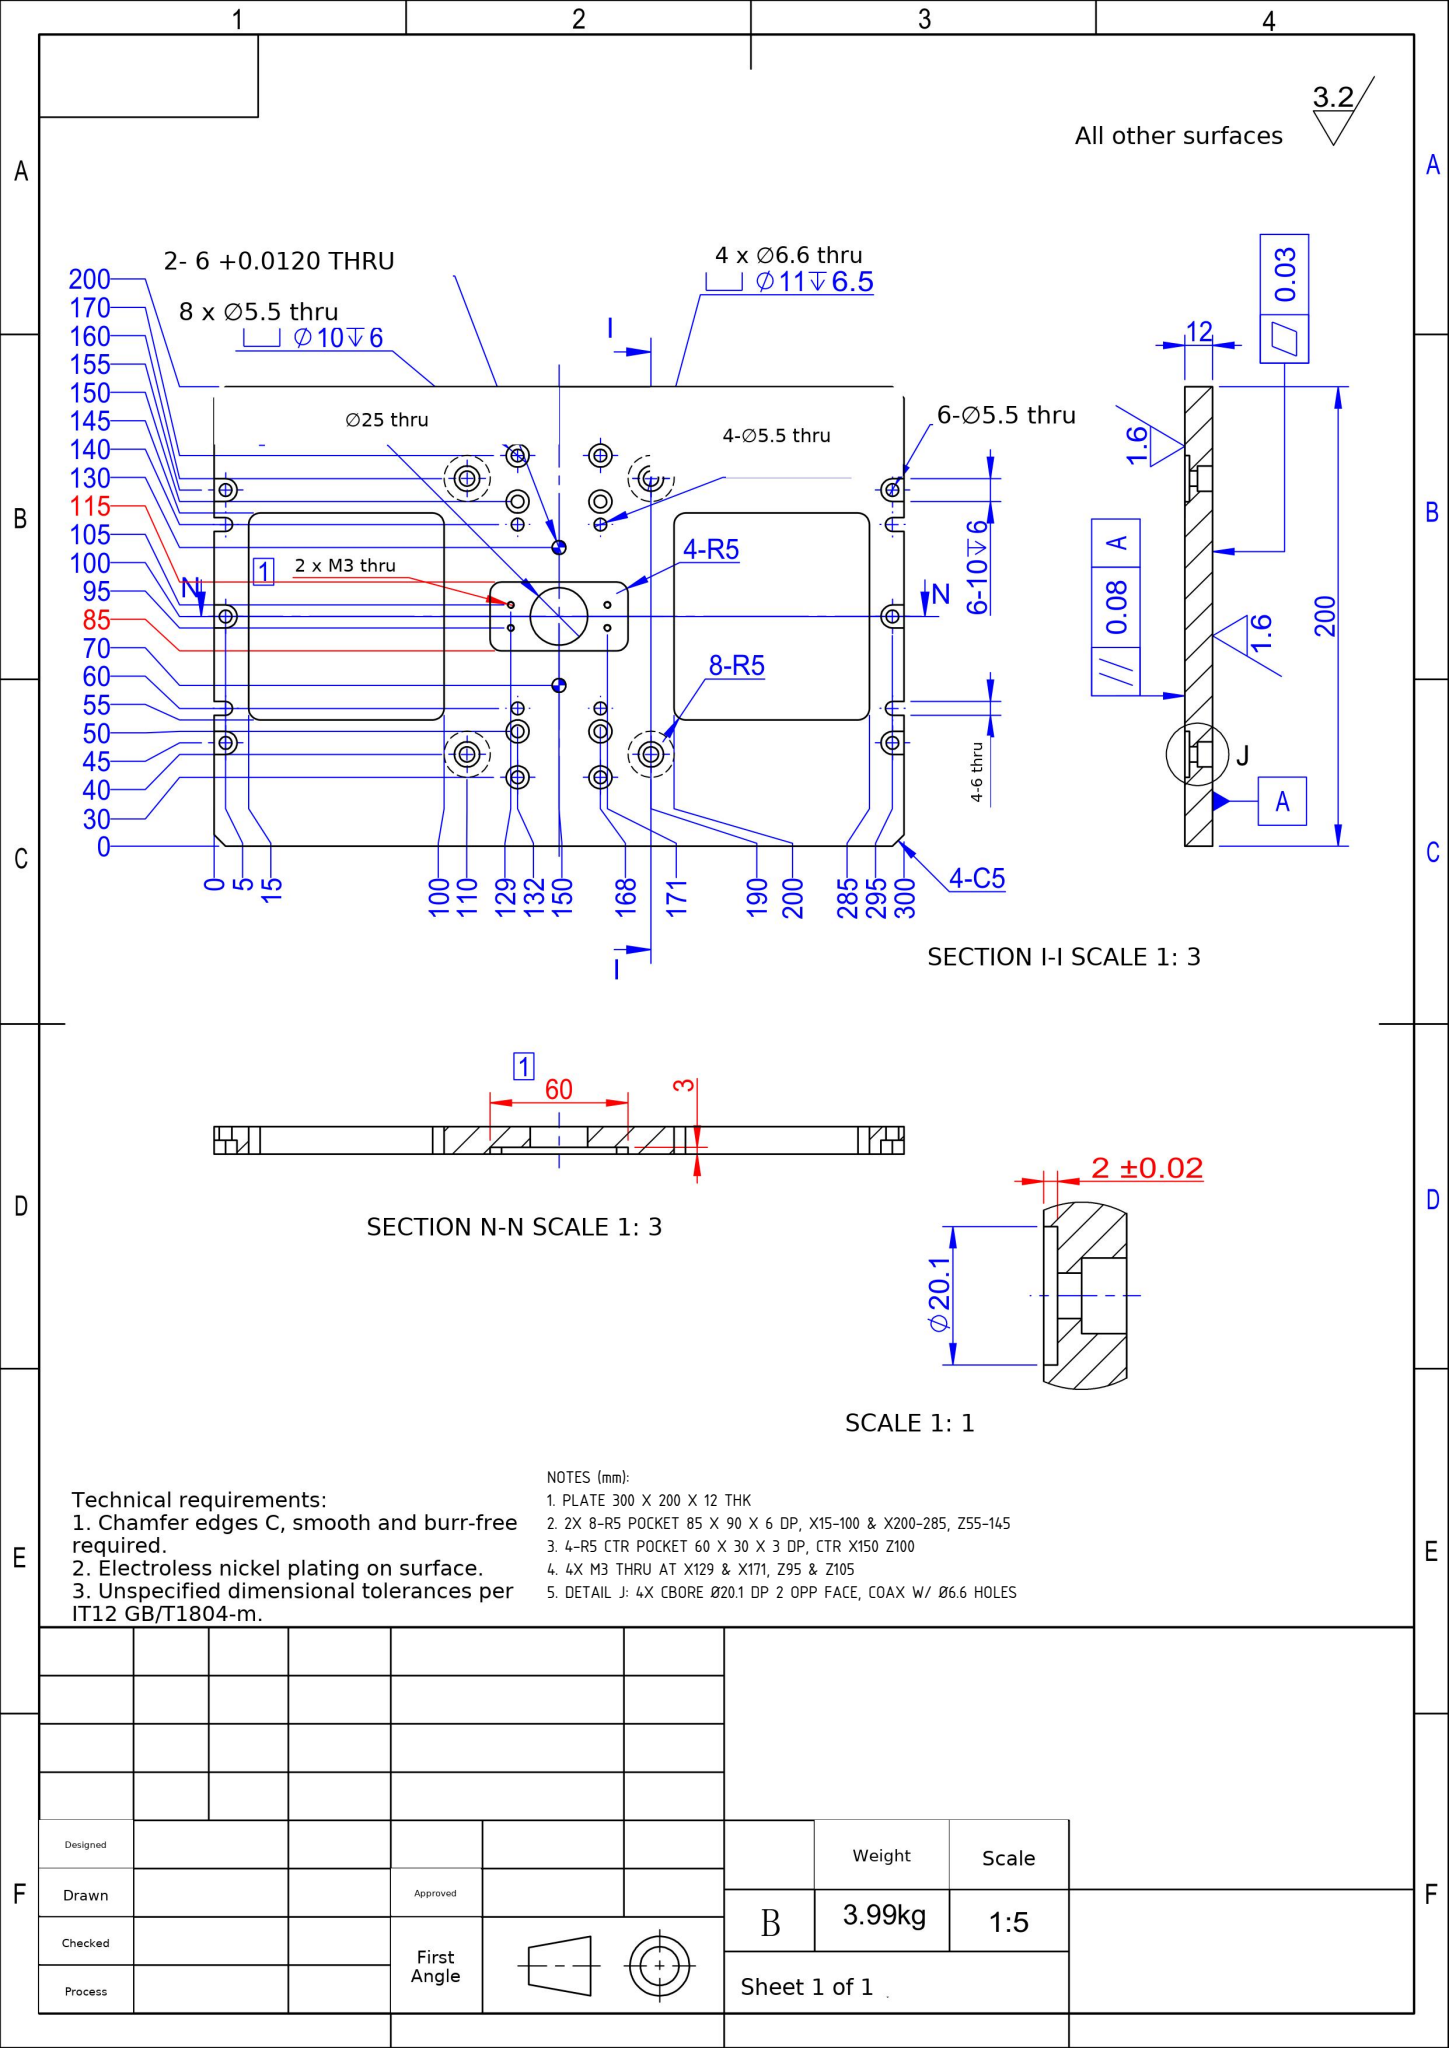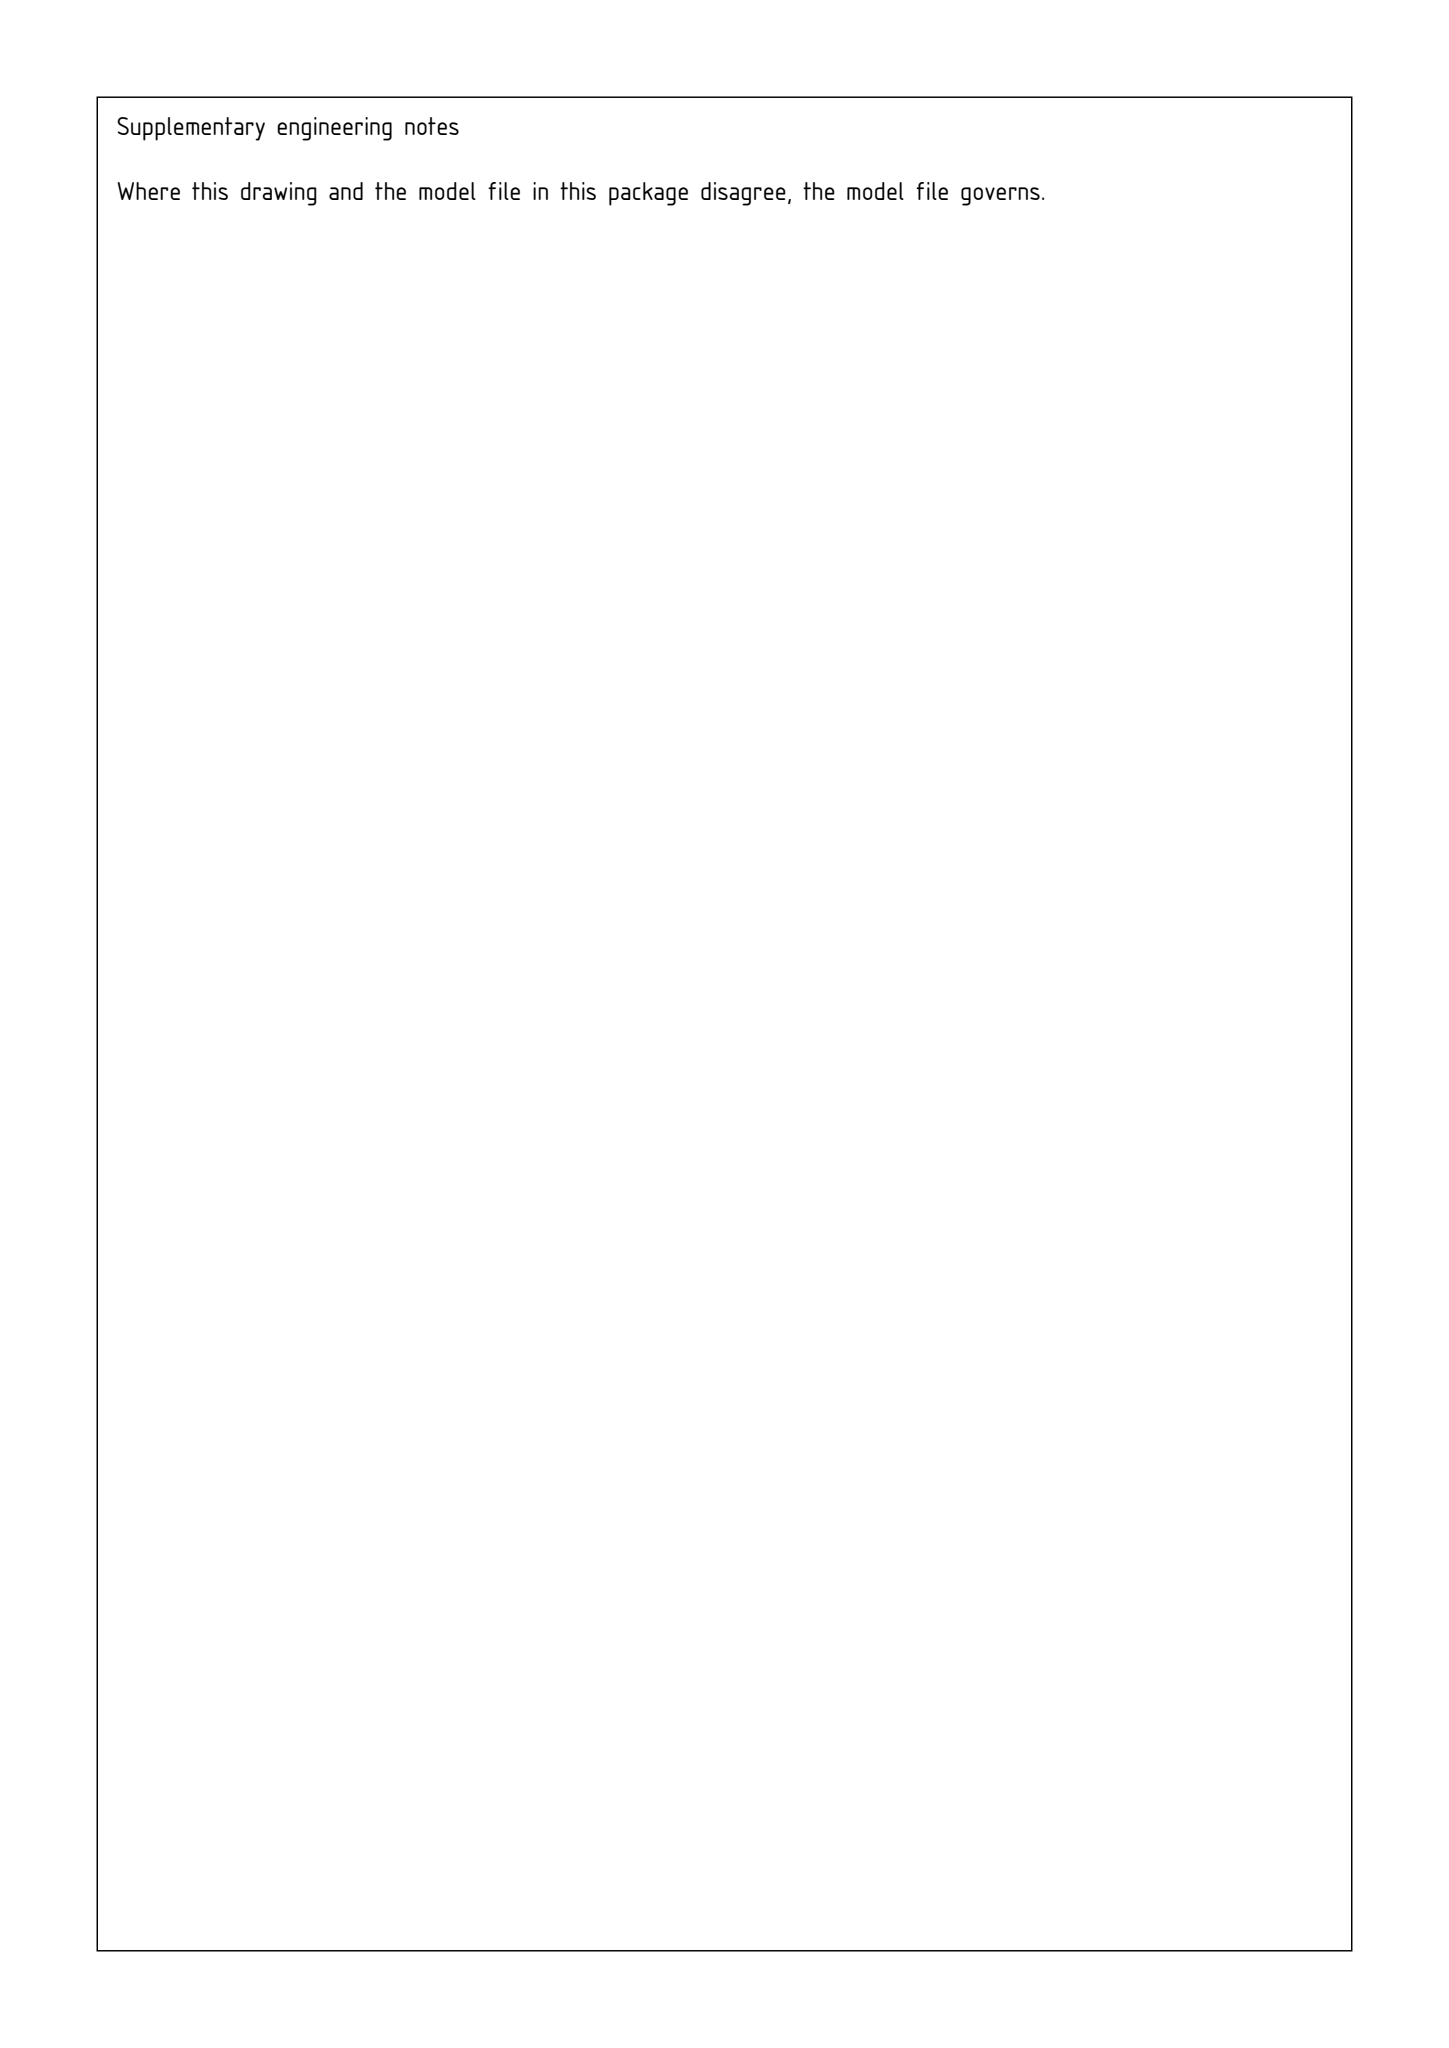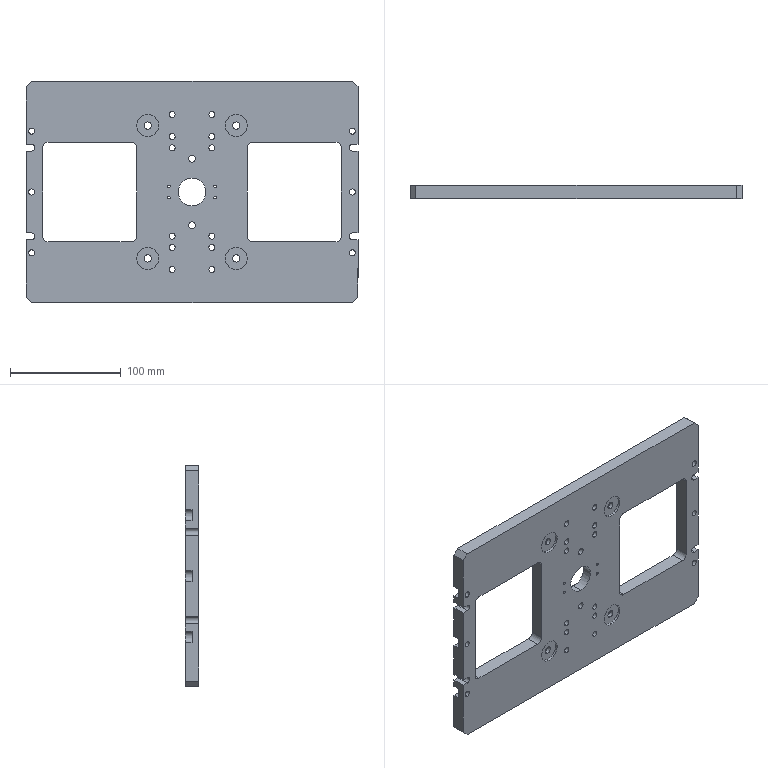Part | SolidWorks | mm | 1 solid | 181 faces | box 300 x 12 x 200 mm | volume 507980 mm3 | cylinder 112 | plane 69 | commonest cylinder face diameters 5.5 x36 10 x34 2.5 x8 6 x8 20.1 x8 11 x8 6.6 x8 25 x2
Drawing notes:
PLATE 300 X 200 X 12 THK | from the solid: bbox_xyz 300 x 12 x 200
2X 8-R5 POCKET 85 X 90 X 6 DP, X15-100 & X200-285, Z55-145 | from the solid: x planes 15/100 & 200/285 (85 wide), z planes 55 & 145 x2 (90), floor y=6 in 12 thk
4-R5 CTR POCKET 60 X 30 X 3 DP, CTR X150 Z100 | from the solid: x planes 120/180 = 60, z planes 85/115 = 30, floor y=9 in 12 thk; O25 bore ctr 150,100
4X M3 THRU AT X129 & X171, Z95 & Z105 | from the solid: O2.5 y-axis holes at (129,95),(129,105),(171,95),(171,105), len 9 thru
DETAIL J: 4X CBORE Ø20.1 DP 2 OPP FACE, COAX W/ Ø6.6 HOLES | from the solid: dia 20.1 len 2 at (110,40),(110,160),(190,40),(190,160); y planes 2.0 x4; same ctrs as Ø6.6/Ø11DP6.5
build123d program:
from build123d import *

# Parameters (mm, degrees)
SKETCH1_W                                       = 300
SKETCH1_H                                       = 200
BOSS_EXTRUDE1_DEPTH                             = 6
SKETCH2_W                                       = 85
SKETCH2_H                                       = 90
CUT_EXTRUDE1_DEPTH                              = 181.677
CHAMFER1_SIZE                                   = 5
M6_HEX_SOCKET_HEAD_CAP_SCREW_CBORE1_D           = 6.6
M6_HEX_SOCKET_HEAD_CAP_SCREW_CBORE1_CBORE_D     = 11
M6_HEX_SOCKET_HEAD_CAP_SCREW_CBORE1_CBORE_DEPTH = 6.5
M5_CLEARANCE_HOLE2_AT_2_COUNT                   = 2
M5_CLEARANCE_HOLE2_AT_2_PITCH                   = 110
M5_CLEARANCE_HOLE2_AT_3_COUNT                   = 2
M5_CLEARANCE_HOLE2_AT_3_PITCH                   = 55
CUT_EXTRUDE10_DEPTH                             = 6
CUT_EXTRUDE11_DEPTH                             = 181.677
FILLET4_R                                       = 5
SKETCH38_R                                      = 10.05
CUT_EXTRUDE9_DEPTH                              = 2
F_6_0_6_DIAMETER_HOLE1_D                        = 6
F_6_0_6_DIAMETER_HOLE1_DEPTH                    = 12
F_6_0_6_DIAMETER_HOLE1_TIP                      = 1.803
M5_HEX_SOCKET_HEAD_CAP_SCREW_CBORE2_D           = 5.5
M5_HEX_SOCKET_HEAD_CAP_SCREW_CBORE2_CBORE_D     = 10
M5_HEX_SOCKET_HEAD_CAP_SCREW_CBORE2_CBORE_DEPTH = 6
F_5_5_5_5_DIAMETER_HOLE1_AT_2_COUNT             = 2
F_5_5_5_5_DIAMETER_HOLE1_AT_2_PITCH             = 80
SKETCH49_R                                      = 12.5
CUT_EXTRUDE12_DEPTH                             = 181.677
M3_TAPPED_HOLE1_D                               = 2.5
SKETCH58_W                                      = 60
SKETCH58_H                                      = 30
CUT_EXTRUDE15_DEPTH                             = 3
FILLET5_R                                       = 5


with BuildPart() as part:
    # Sketch1 → Boss-Extrude1 (new, symmetric)
    with BuildSketch(Plane(origin=(0, 0, 0), x_dir=(1, 0, 0), z_dir=(0, 1, 0))):
        Rectangle(SKETCH1_W, SKETCH1_H)
    extrude(amount=BOSS_EXTRUDE1_DEPTH, both=True)

    # Sketch2 → Cut-Extrude1 (cut, through all)
    with BuildSketch(Plane(origin=(0, 6, 0), x_dir=(1, 0, 0), z_dir=(0, 1, 0))):
        with Locations((-92.5, 0)):
            Rectangle(SKETCH2_W, SKETCH2_H)
    cut_extrude1 = extrude(amount=-CUT_EXTRUDE1_DEPTH, mode=Mode.SUBTRACT)

    # Mirror1: Cut-Extrude1 across plane
    add(cut_extrude1.mirror(Plane(origin=(0, 0, 0), x_dir=(0, 0, 1), z_dir=(1, 0, 0))), mode=Mode.SUBTRACT)

    # Chamfer1
    chamfer1_edges = [part.edges().sort_by_distance(p)[0] for p in [
        (-150, 0, -100),
        (150, 0, -100),
        (150, 0, 100),
        (-150, 0, 100),
    ]]
    chamfer(chamfer1_edges, length=CHAMFER1_SIZE)

    # M6 Hex Socket Head Cap Screw CBORE1 (through all)
    with Locations(Plane(origin=(0, 6, 0), x_dir=(-1, 0, 0), z_dir=(0, 1, 0))):
        with Locations((40, -60), (-40, -60), (-40, 60), (40, 60)):
            CounterBoreHole(M6_HEX_SOCKET_HEAD_CAP_SCREW_CBORE1_D / 2, M6_HEX_SOCKET_HEAD_CAP_SCREW_CBORE1_CBORE_D / 2, M6_HEX_SOCKET_HEAD_CAP_SCREW_CBORE1_CBORE_DEPTH)

    # Sketch32 → M5 Clearance Hole2 (revolve, cut)
    with BuildSketch(Plane(origin=(-145, 6, 55), x_dir=(0, 0, 1), z_dir=(1, 0, 0))):
        Polygon((0, 0), (0, 13.652), (2.75, 12), (2.75, 0), align=None)
    m5_clearance_hole2 = revolve(axis=Axis((-145, 12.35, 55), (0, -1, 0)), mode=Mode.SUBTRACT)

    # M5 Clearance Hole2 at 2: M5 Clearance Hole2 ×2
    with Locations(*[(0, 0, -i * M5_CLEARANCE_HOLE2_AT_2_PITCH) for i in range(1, M5_CLEARANCE_HOLE2_AT_2_COUNT)]):
        add(m5_clearance_hole2, mode=Mode.SUBTRACT)

    # M5 Clearance Hole2 at 3: M5 Clearance Hole2 ×2
    with Locations(*[(0, 0, -i * M5_CLEARANCE_HOLE2_AT_3_PITCH) for i in range(1, M5_CLEARANCE_HOLE2_AT_3_COUNT)]):
        add(m5_clearance_hole2, mode=Mode.SUBTRACT)

    # Sketch39 → Cut-Extrude10 (cut)
    with BuildSketch(Plane(origin=(0, 6, 0), x_dir=(1, 0, 0), z_dir=(0, 1, 0))):
        with BuildLine():
            Line((-145, 50), (-150, 50))
            ThreePointArc((-150, 50), (-155, 55), (-150, 60))
            Line((-150, 60), (-145, 60))
            ThreePointArc((-145, 60), (-140, 55), (-145, 50))
        make_face()
        with BuildLine():
            Line((-145, -5), (-150, -5))
            ThreePointArc((-150, -5), (-155, 0), (-150, 5))
            Line((-150, 5), (-145, 5))
            ThreePointArc((-145, 5), (-140, 0), (-145, -5))
        make_face()
        with BuildLine():
            Line((-145, -60), (-150, -60))
            ThreePointArc((-150, -60), (-155, -55), (-150, -50))
            Line((-150, -50), (-145, -50))
            ThreePointArc((-145, -50), (-140, -55), (-145, -60))
        make_face()
    cut_extrude10 = extrude(amount=-CUT_EXTRUDE10_DEPTH, mode=Mode.SUBTRACT)

    # Sketch40 → Cut-Extrude11 (cut, through all)
    with BuildSketch(Plane(origin=(0, 6, 0), x_dir=(1, 0, 0), z_dir=(0, 1, 0))):
        with BuildLine():
            Line((-150, 43), (-145, 43))
            ThreePointArc((-145, 43), (-142, 40), (-145, 37))
            Line((-145, 37), (-150, 37))
            ThreePointArc((-150, 37), (-153, 40), (-150, 43))
        make_face()
        with BuildLine():
            Line((-150, -37), (-145, -37))
            ThreePointArc((-145, -37), (-142, -40), (-145, -43))
            Line((-145, -43), (-150, -43))
            ThreePointArc((-150, -43), (-153, -40), (-150, -37))
        make_face()
    cut_extrude11 = extrude(amount=-CUT_EXTRUDE11_DEPTH, mode=Mode.SUBTRACT)

    # Mirror15: M5 Clearance Hole2, Cut-Extrude10, Cut-Extrude11 across plane
    add(m5_clearance_hole2.mirror(Plane(origin=(0, 0, 0), x_dir=(0, 0, 1), z_dir=(1, 0, 0))), mode=Mode.SUBTRACT)
    add(cut_extrude10.mirror(Plane(origin=(0, 0, 0), x_dir=(0, 0, 1), z_dir=(1, 0, 0))), mode=Mode.SUBTRACT)
    add(cut_extrude11.mirror(Plane(origin=(0, 0, 0), x_dir=(0, 0, 1), z_dir=(1, 0, 0))), mode=Mode.SUBTRACT)

    # Mirror15 copy 1 sketch → Mirror15 copy 1 (revolve, cut)
    with BuildSketch(Plane(origin=(145, 6, -55), x_dir=(0, 0, 1), z_dir=(-1, 0, 0))):
        Polygon((0, 0), (0, -13.652), (2.75, -12), (2.75, 0), align=None)
    revolve(axis=Axis((145, 12.35, -55), (0, 1, 0)), mode=Mode.SUBTRACT)

    # Mirror15 copy 2 sketch → Mirror15 copy 2 (revolve, cut)
    with BuildSketch(Plane(origin=(145, 6, 0), x_dir=(0, 0, 1), z_dir=(-1, 0, 0))):
        Polygon((0, 0), (0, -13.652), (2.75, -12), (2.75, 0), align=None)
    revolve(axis=Axis((145, 12.35, 0), (0, 1, 0)), mode=Mode.SUBTRACT)

    # Fillet4
    fillet4_edges = [part.edges().sort_by_distance(p)[0] for p in [
        (-135, 0, 45),
        (-135, 0, -45),
        (-50, 0, -45),
        (-50, 0, 45),
        (135, 0, -45),
        (135, 0, 45),
        (50, 0, 45),
        (50, 0, -45),
    ]]
    fillet(fillet4_edges, radius=FILLET4_R)

    # Sketch38 → Cut-Extrude9 (cut)
    with BuildSketch(Plane.XZ.offset(6)):
        with Locations(Location((-40, 60, 0), (0, 0, 270))):
            Circle(SKETCH38_R)
        with Locations(Location((40, 60, 0), (0, 0, 270))):
            Circle(SKETCH38_R)
        with Locations(Location((40, -60, 0), (0, 0, 270))):
            Circle(SKETCH38_R)
        with Locations(Location((-40, -60, 0), (0, 0, 270))):
            Circle(SKETCH38_R)
    extrude(amount=-CUT_EXTRUDE9_DEPTH, mode=Mode.SUBTRACT)

    # 6.0 _6_ Diameter Hole1
    with Locations(Plane(origin=(0, 6, 0), x_dir=(-1, 0, 0), z_dir=(0, 1, 0))):
        with Locations((0, -30), (0, 30)):
            Hole(F_6_0_6_DIAMETER_HOLE1_D / 2, depth=F_6_0_6_DIAMETER_HOLE1_DEPTH)
            with Locations((0, 0, -(F_6_0_6_DIAMETER_HOLE1_DEPTH + F_6_0_6_DIAMETER_HOLE1_TIP / 2))):  # 118° drill point
                Cone(0, F_6_0_6_DIAMETER_HOLE1_D / 2, F_6_0_6_DIAMETER_HOLE1_TIP, mode=Mode.SUBTRACT)

    # M5 Hex Socket Head Cap Screw CBORE2 (through all)
    with Locations(Plane(origin=(0, 6, 0), x_dir=(-1, 0, 0), z_dir=(0, 1, 0))):
        with Locations((18, -70), (18, 70), (18, -50), (18, 50)):
            m5_hex_socket_head_cap_screw_cbore2 = CounterBoreHole(M5_HEX_SOCKET_HEAD_CAP_SCREW_CBORE2_D / 2, M5_HEX_SOCKET_HEAD_CAP_SCREW_CBORE2_CBORE_D / 2, M5_HEX_SOCKET_HEAD_CAP_SCREW_CBORE2_CBORE_DEPTH)

    # Sketch47 → 5.5 _5.5_ Diameter Hole1 (revolve, cut)
    with BuildSketch(Plane(origin=(-18, 6, -40), x_dir=(0, 0, 1), z_dir=(1, 0, 0))):
        Polygon((0, 0), (0, 13.652), (2.75, 12), (2.75, 0), align=None)
    f_5_5_5_5_diameter_hole1 = revolve(axis=Axis((-18, 12.35, -40), (0, -1, 0)), mode=Mode.SUBTRACT)

    # 5.5 _5.5_ Diameter Hole1 at 2: 5.5 _5.5_ Diameter Hole1 ×2
    with Locations(*[(0, 0, i * F_5_5_5_5_DIAMETER_HOLE1_AT_2_PITCH) for i in range(1, F_5_5_5_5_DIAMETER_HOLE1_AT_2_COUNT)]):
        add(f_5_5_5_5_diameter_hole1, mode=Mode.SUBTRACT)

    # Mirror18: M5 Hex Socket Head Cap Screw CBORE2, 5.5 _5.5_ Diameter Hole1 across plane
    add(m5_hex_socket_head_cap_screw_cbore2.mirror(Plane(origin=(0, 0, 0), x_dir=(0, 0, 1), z_dir=(1, 0, 0))), mode=Mode.SUBTRACT)
    add(f_5_5_5_5_diameter_hole1.mirror(Plane(origin=(0, 0, 0), x_dir=(0, 0, 1), z_dir=(1, 0, 0))), mode=Mode.SUBTRACT)

    # Mirror18 copy 1 sketch → Mirror18 copy 1 (revolve, cut)
    with BuildSketch(Plane(origin=(18, 6, 40), x_dir=(0, 0, 1), z_dir=(-1, 0, 0))):
        Polygon((0, 0), (0, -13.652), (2.75, -12), (2.75, 0), align=None)
    revolve(axis=Axis((18, 12.35, 40), (0, 1, 0)), mode=Mode.SUBTRACT)

    # Sketch49 → Cut-Extrude12 (cut, through all)
    with BuildSketch(Plane(origin=(0, 6, 0), x_dir=(1, 0, 0), z_dir=(0, 1, 0))):
        with Locations(Location((0, 0, 0), (0, 0, 270))):
            Circle(SKETCH49_R)
    extrude(amount=-CUT_EXTRUDE12_DEPTH, mode=Mode.SUBTRACT)

    # M3 Tapped Hole1 (through all)
    with Locations(Plane(origin=(27.337, -6, 7.727), x_dir=(-1, 0, 0), z_dir=(0, -1, 0))):
        with Locations((48.337, 12.727), (48.337, 2.727)):
            m3_tapped_hole1 = Hole(M3_TAPPED_HOLE1_D / 2)

    # Mirror19: M3 Tapped Hole1 across plane
    add(m3_tapped_hole1.mirror(Plane(origin=(0, 0, 0), x_dir=(0, 0, 1), z_dir=(1, 0, 0))), mode=Mode.SUBTRACT)

    # Sketch58 → Cut-Extrude15 (cut)
    with BuildSketch(Plane(origin=(0, 6, 0), x_dir=(1, 0, 0), z_dir=(0, 1, 0))):
        Rectangle(SKETCH58_W, SKETCH58_H)
    extrude(amount=-CUT_EXTRUDE15_DEPTH, mode=Mode.SUBTRACT)

    # Fillet5
    fillet5_edges = [part.edges().sort_by_distance(p)[0] for p in [
        (30, 4.5, -15),
        (30, 4.5, 15),
        (-30, 4.5, 15),
        (-30, 4.5, -15),
    ]]
    fillet(fillet5_edges, radius=FILLET5_R)


solid = part.part